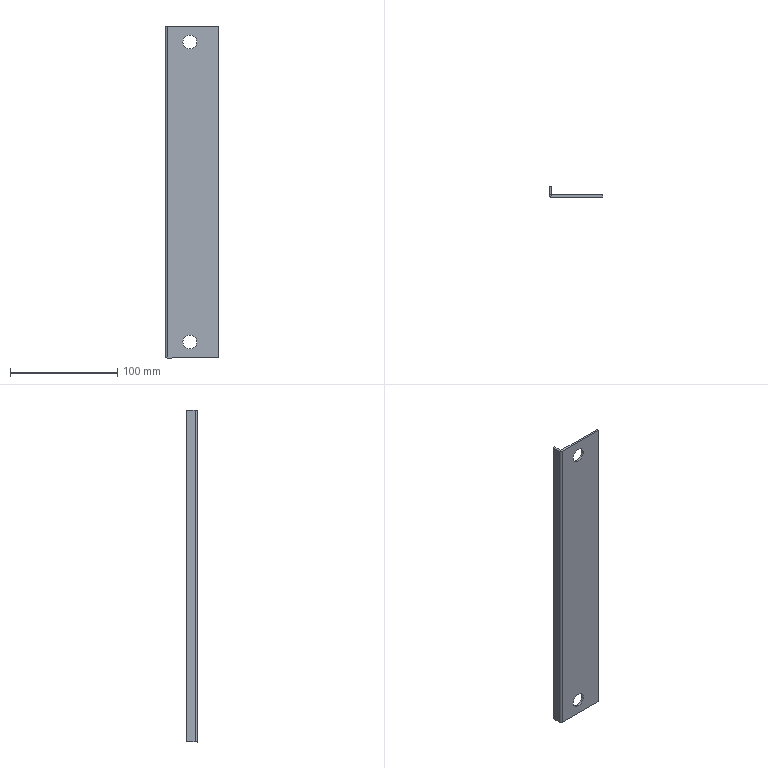Component | SolidWorks | BottomPlateReinforcementBeam-1 | 1 solid | 18 faces | box 50 x 10 x 310 mm | volume 35136 mm3 | plane 12 | cylinder 6 | commonest cylinder face diameters 13 x4 4.2 x1 0.2 x1
STEP:
#1=COLOUR_RGB('',0.7922,0.8196,0.9333);
#2=FILL_AREA_STYLE_COLOUR('',#1);
#3=FILL_AREA_STYLE('',(#2));
#4=SURFACE_STYLE_FILL_AREA(#3);
#5=SURFACE_SIDE_STYLE('',(#4));
#6=SURFACE_STYLE_USAGE(.BOTH.,#5);
#7=PRESENTATION_STYLE_ASSIGNMENT((#6));
#8=CARTESIAN_POINT('',(-12.829,-17.663,36.708));
#9=VERTEX_POINT('',#8);
#10=CARTESIAN_POINT('',(-12.317,-17.663,36.708));
#11=VERTEX_POINT('',#10);
#12=CARTESIAN_POINT('',(-12.573,-17.663,36.708));
#13=DIRECTION('',(0.,1.,-0.));
#14=DIRECTION('',(1.,-0.,0.));
#15=AXIS2_PLACEMENT_3D('',#12,#13,#14);
#16=CIRCLE('',#15,0.2559);
#17=EDGE_CURVE('',#9,#11,#16,.T.);
#18=ORIENTED_EDGE('',*,*,#17,.F.);
#19=CARTESIAN_POINT('',(-12.829,-17.584,36.708));
#20=VERTEX_POINT('',#19);
#21=CARTESIAN_POINT('',(-12.829,-17.978,36.708));
#22=DIRECTION('',(0.,1.,-0.));
#23=VECTOR('',#22,39.37);
#24=LINE('',#21,#23);
#25=EDGE_CURVE('',#9,#20,#24,.T.);
#26=ORIENTED_EDGE('',*,*,#25,.T.);
#27=CARTESIAN_POINT('',(-12.317,-17.584,36.708));
#28=VERTEX_POINT('',#27);
#29=CARTESIAN_POINT('',(-12.573,-17.584,36.708));
#30=DIRECTION('',(0.,1.,-0.));
#31=DIRECTION('',(1.,-0.,0.));
#32=AXIS2_PLACEMENT_3D('',#29,#30,#31);
#33=CIRCLE('',#32,0.2559);
#34=EDGE_CURVE('',#20,#28,#33,.T.);
#35=ORIENTED_EDGE('',*,*,#34,.T.);
#36=CARTESIAN_POINT('',(-12.317,-17.978,36.708));
#37=DIRECTION('',(0.,1.,-0.));
#38=VECTOR('',#37,39.37);
#39=LINE('',#36,#38);
#40=EDGE_CURVE('',#11,#28,#39,.T.);
#41=ORIENTED_EDGE('',*,*,#40,.F.);
#42=EDGE_LOOP('',(#18,#26,#35,#41));
#43=FACE_OUTER_BOUND('',#42,.T.);
#44=CARTESIAN_POINT('',(-12.573,-17.978,36.708));
#45=DIRECTION('',(0.,1.,-0.));
#46=DIRECTION('',(1.,-0.,0.));
#47=AXIS2_PLACEMENT_3D('',#44,#45,#46);
#48=CYLINDRICAL_SURFACE('',#47,0.2559);
#49=ADVANCED_FACE('',(#43),#48,.F.);
#50=CARTESIAN_POINT('',(-12.829,-17.663,25.685));
#51=VERTEX_POINT('',#50);
#52=CARTESIAN_POINT('',(-12.317,-17.663,25.685));
#53=VERTEX_POINT('',#52);
#54=CARTESIAN_POINT('',(-12.573,-17.663,25.685));
#55=DIRECTION('',(0.,1.,-0.));
#56=DIRECTION('',(1.,-0.,0.));
#57=AXIS2_PLACEMENT_3D('',#54,#55,#56);
#58=CIRCLE('',#57,0.2559);
#59=EDGE_CURVE('',#51,#53,#58,.T.);
#60=ORIENTED_EDGE('',*,*,#59,.F.);
#61=CARTESIAN_POINT('',(-12.829,-17.584,25.685));
#62=VERTEX_POINT('',#61);
#63=CARTESIAN_POINT('',(-12.829,-17.978,25.685));
#64=DIRECTION('',(0.,1.,-0.));
#65=VECTOR('',#64,39.37);
#66=LINE('',#63,#65);
#67=EDGE_CURVE('',#51,#62,#66,.T.);
#68=ORIENTED_EDGE('',*,*,#67,.T.);
#69=CARTESIAN_POINT('',(-12.317,-17.584,25.685));
#70=VERTEX_POINT('',#69);
#71=CARTESIAN_POINT('',(-12.573,-17.584,25.685));
#72=DIRECTION('',(0.,1.,-0.));
#73=DIRECTION('',(1.,-0.,0.));
#74=AXIS2_PLACEMENT_3D('',#71,#72,#73);
#75=CIRCLE('',#74,0.2559);
#76=EDGE_CURVE('',#62,#70,#75,.T.);
#77=ORIENTED_EDGE('',*,*,#76,.T.);
#78=CARTESIAN_POINT('',(-12.317,-17.978,25.685));
#79=DIRECTION('',(0.,1.,-0.));
#80=VECTOR('',#79,39.37);
#81=LINE('',#78,#80);
#82=EDGE_CURVE('',#53,#70,#81,.T.);
#83=ORIENTED_EDGE('',*,*,#82,.F.);
#84=EDGE_LOOP('',(#60,#68,#77,#83));
#85=FACE_OUTER_BOUND('',#84,.T.);
#86=CARTESIAN_POINT('',(-12.573,-17.978,25.685));
#87=DIRECTION('',(0.,1.,-0.));
#88=DIRECTION('',(1.,-0.,0.));
#89=AXIS2_PLACEMENT_3D('',#86,#87,#88);
#90=CYLINDRICAL_SURFACE('',#89,0.2559);
#91=ADVANCED_FACE('',(#85),#90,.F.);
#92=CARTESIAN_POINT('',(-13.396,-17.584,37.299));
#93=VERTEX_POINT('',#92);
#94=CARTESIAN_POINT('',(-11.51,-17.584,37.299));
#95=VERTEX_POINT('',#94);
#96=CARTESIAN_POINT('',(-13.479,-17.584,37.299));
#97=DIRECTION('',(1.,-0.,0.));
#98=VECTOR('',#97,39.37);
#99=LINE('',#96,#98);
#100=EDGE_CURVE('',#93,#95,#99,.T.);
#101=ORIENTED_EDGE('',*,*,#100,.F.);
#102=CARTESIAN_POINT('',(-13.396,-17.663,37.299));
#103=VERTEX_POINT('',#102);
#104=CARTESIAN_POINT('',(-13.396,-17.584,37.299));
#105=DIRECTION('',(0.,-1.,0.));
#106=VECTOR('',#105,39.37);
#107=LINE('',#104,#106);
#108=EDGE_CURVE('',#93,#103,#107,.T.);
#109=ORIENTED_EDGE('',*,*,#108,.T.);
#110=CARTESIAN_POINT('',(-11.51,-17.663,37.299));
#111=VERTEX_POINT('',#110);
#112=CARTESIAN_POINT('',(-13.479,-17.663,37.299));
#113=DIRECTION('',(1.,-0.,0.));
#114=VECTOR('',#113,39.37);
#115=LINE('',#112,#114);
#116=EDGE_CURVE('',#103,#111,#115,.T.);
#117=ORIENTED_EDGE('',*,*,#116,.T.);
#118=CARTESIAN_POINT('',(-11.51,-17.663,37.299));
#119=DIRECTION('',(0.,1.,-0.));
#120=VECTOR('',#119,39.37);
#121=LINE('',#118,#120);
#122=EDGE_CURVE('',#111,#95,#121,.T.);
#123=ORIENTED_EDGE('',*,*,#122,.T.);
#124=EDGE_LOOP('',(#101,#109,#117,#123));
#125=FACE_OUTER_BOUND('',#124,.T.);
#126=CARTESIAN_POINT('',(-13.479,-17.663,37.299));
#127=DIRECTION('',(-0.,0.,1.));
#128=DIRECTION('',(-0.,-1.,0.));
#129=AXIS2_PLACEMENT_3D('',#126,#127,#128);
#130=PLANE('',#129);
#131=ADVANCED_FACE('',(#125),#130,.T.);
#132=CARTESIAN_POINT('',(-12.573,-17.663,25.685));
#133=DIRECTION('',(0.,1.,-0.));
#134=DIRECTION('',(1.,-0.,0.));
#135=AXIS2_PLACEMENT_3D('',#132,#133,#134);
#136=CIRCLE('',#135,0.2559);
#137=EDGE_CURVE('',#53,#51,#136,.T.);
#138=ORIENTED_EDGE('',*,*,#137,.T.);
#139=ORIENTED_EDGE('',*,*,#59,.T.);
#140=EDGE_LOOP('',(#138,#139));
#141=FACE_BOUND('',#140,.T.);
#142=CARTESIAN_POINT('',(-12.573,-17.663,36.708));
#143=DIRECTION('',(0.,1.,-0.));
#144=DIRECTION('',(1.,-0.,0.));
#145=AXIS2_PLACEMENT_3D('',#142,#143,#144);
#146=CIRCLE('',#145,0.2559);
#147=EDGE_CURVE('',#11,#9,#146,.T.);
#148=ORIENTED_EDGE('',*,*,#147,.T.);
#149=ORIENTED_EDGE('',*,*,#17,.T.);
#150=EDGE_LOOP('',(#148,#149));
#151=FACE_BOUND('',#150,.T.);
#152=CARTESIAN_POINT('',(-13.396,-17.663,25.094));
#153=VERTEX_POINT('',#152);
#154=CARTESIAN_POINT('',(-13.396,-17.663,37.299));
#155=DIRECTION('',(0.,-0.,-1.));
#156=VECTOR('',#155,39.37);
#157=LINE('',#154,#156);
#158=EDGE_CURVE('',#103,#153,#157,.T.);
#159=ORIENTED_EDGE('',*,*,#158,.T.);
#160=CARTESIAN_POINT('',(-11.51,-17.663,25.094));
#161=VERTEX_POINT('',#160);
#162=CARTESIAN_POINT('',(-13.479,-17.663,25.094));
#163=DIRECTION('',(-1.,0.,-0.));
#164=VECTOR('',#163,39.37);
#165=LINE('',#162,#164);
#166=EDGE_CURVE('',#161,#153,#165,.T.);
#167=ORIENTED_EDGE('',*,*,#166,.F.);
#168=CARTESIAN_POINT('',(-11.51,-17.663,25.094));
#169=DIRECTION('',(0.,-0.,-1.));
#170=VECTOR('',#169,39.37);
#171=LINE('',#168,#170);
#172=EDGE_CURVE('',#111,#161,#171,.T.);
#173=ORIENTED_EDGE('',*,*,#172,.F.);
#174=ORIENTED_EDGE('',*,*,#116,.F.);
#175=EDGE_LOOP('',(#159,#167,#173,#174));
#176=FACE_OUTER_BOUND('',#175,.T.);
#177=CARTESIAN_POINT('',(-12.494,-17.663,31.196));
#178=DIRECTION('',(0.,1.,-0.));
#179=DIRECTION('',(1.,-0.,0.));
#180=AXIS2_PLACEMENT_3D('',#177,#178,#179);
#181=PLANE('',#180);
#182=ADVANCED_FACE('',(#141,#151,#176),#181,.F.);
#183=CARTESIAN_POINT('',(-12.573,-17.584,36.708));
#184=DIRECTION('',(0.,1.,-0.));
#185=DIRECTION('',(1.,-0.,0.));
#186=AXIS2_PLACEMENT_3D('',#183,#184,#185);
#187=CIRCLE('',#186,0.2559);
#188=EDGE_CURVE('',#28,#20,#187,.T.);
#189=ORIENTED_EDGE('',*,*,#188,.F.);
#190=ORIENTED_EDGE('',*,*,#34,.F.);
#191=EDGE_LOOP('',(#189,#190));
#192=FACE_BOUND('',#191,.T.);
#193=CARTESIAN_POINT('',(-12.573,-17.584,25.685));
#194=DIRECTION('',(0.,1.,-0.));
#195=DIRECTION('',(1.,-0.,0.));
#196=AXIS2_PLACEMENT_3D('',#193,#194,#195);
#197=CIRCLE('',#196,0.2559);
#198=EDGE_CURVE('',#70,#62,#197,.T.);
#199=ORIENTED_EDGE('',*,*,#198,.F.);
#200=ORIENTED_EDGE('',*,*,#76,.F.);
#201=EDGE_LOOP('',(#199,#200));
#202=FACE_BOUND('',#201,.T.);
#203=CARTESIAN_POINT('',(-11.51,-17.584,25.094));
#204=VERTEX_POINT('',#203);
#205=CARTESIAN_POINT('',(-13.396,-17.584,25.094));
#206=VERTEX_POINT('',#205);
#207=CARTESIAN_POINT('',(-13.479,-17.584,25.094));
#208=DIRECTION('',(-1.,0.,-0.));
#209=VECTOR('',#208,39.37);
#210=LINE('',#207,#209);
#211=EDGE_CURVE('',#204,#206,#210,.T.);
#212=ORIENTED_EDGE('',*,*,#211,.T.);
#213=CARTESIAN_POINT('',(-13.396,-17.584,37.299));
#214=DIRECTION('',(0.,-0.,-1.));
#215=VECTOR('',#214,39.37);
#216=LINE('',#213,#215);
#217=EDGE_CURVE('',#93,#206,#216,.T.);
#218=ORIENTED_EDGE('',*,*,#217,.F.);
#219=ORIENTED_EDGE('',*,*,#100,.T.);
#220=CARTESIAN_POINT('',(-11.51,-17.584,25.094));
#221=DIRECTION('',(0.,-0.,-1.));
#222=VECTOR('',#221,39.37);
#223=LINE('',#220,#222);
#224=EDGE_CURVE('',#95,#204,#223,.T.);
#225=ORIENTED_EDGE('',*,*,#224,.T.);
#226=EDGE_LOOP('',(#212,#218,#219,#225));
#227=FACE_OUTER_BOUND('',#226,.T.);
#228=CARTESIAN_POINT('',(-12.494,-17.584,31.196));
#229=DIRECTION('',(0.,1.,-0.));
#230=DIRECTION('',(1.,-0.,0.));
#231=AXIS2_PLACEMENT_3D('',#228,#229,#230);
#232=PLANE('',#231);
#233=ADVANCED_FACE('',(#192,#202,#227),#232,.T.);
#234=ORIENTED_EDGE('',*,*,#224,.F.);
#235=ORIENTED_EDGE('',*,*,#122,.F.);
#236=ORIENTED_EDGE('',*,*,#172,.T.);
#237=CARTESIAN_POINT('',(-11.51,-17.663,25.094));
#238=DIRECTION('',(0.,1.,-0.));
#239=VECTOR('',#238,39.37);
#240=LINE('',#237,#239);
#241=EDGE_CURVE('',#161,#204,#240,.T.);
#242=ORIENTED_EDGE('',*,*,#241,.T.);
#243=EDGE_LOOP('',(#234,#235,#236,#242));
#244=FACE_OUTER_BOUND('',#243,.T.);
#245=CARTESIAN_POINT('',(-11.51,-17.663,25.094));
#246=DIRECTION('',(1.,-0.,0.));
#247=DIRECTION('',(0.,-0.,-1.));
#248=AXIS2_PLACEMENT_3D('',#245,#246,#247);
#249=PLANE('',#248);
#250=ADVANCED_FACE('',(#244),#249,.T.);
#251=CARTESIAN_POINT('',(-13.396,-17.584,25.094));
#252=DIRECTION('',(0.,-1.,0.));
#253=VECTOR('',#252,39.37);
#254=LINE('',#251,#253);
#255=EDGE_CURVE('',#206,#153,#254,.T.);
#256=ORIENTED_EDGE('',*,*,#255,.F.);
#257=ORIENTED_EDGE('',*,*,#211,.F.);
#258=ORIENTED_EDGE('',*,*,#241,.F.);
#259=ORIENTED_EDGE('',*,*,#166,.T.);
#260=EDGE_LOOP('',(#256,#257,#258,#259));
#261=FACE_OUTER_BOUND('',#260,.T.);
#262=CARTESIAN_POINT('',(-13.479,-17.663,25.094));
#263=DIRECTION('',(0.,-0.,-1.));
#264=DIRECTION('',(0.,1.,-0.));
#265=AXIS2_PLACEMENT_3D('',#262,#263,#264);
#266=PLANE('',#265);
#267=ADVANCED_FACE('',(#261),#266,.T.);
#268=ORIENTED_EDGE('',*,*,#67,.F.);
#269=ORIENTED_EDGE('',*,*,#137,.F.);
#270=ORIENTED_EDGE('',*,*,#82,.T.);
#271=ORIENTED_EDGE('',*,*,#198,.T.);
#272=EDGE_LOOP('',(#268,#269,#270,#271));
#273=FACE_OUTER_BOUND('',#272,.T.);
#274=CARTESIAN_POINT('',(-12.573,-17.978,25.685));
#275=DIRECTION('',(0.,1.,-0.));
#276=DIRECTION('',(1.,-0.,0.));
#277=AXIS2_PLACEMENT_3D('',#274,#275,#276);
#278=CYLINDRICAL_SURFACE('',#277,0.2559);
#279=ADVANCED_FACE('',(#273),#278,.F.);
#280=ORIENTED_EDGE('',*,*,#25,.F.);
#281=ORIENTED_EDGE('',*,*,#147,.F.);
#282=ORIENTED_EDGE('',*,*,#40,.T.);
#283=ORIENTED_EDGE('',*,*,#188,.T.);
#284=EDGE_LOOP('',(#280,#281,#282,#283));
#285=FACE_OUTER_BOUND('',#284,.T.);
#286=CARTESIAN_POINT('',(-12.573,-17.978,36.708));
#287=DIRECTION('',(0.,1.,-0.));
#288=DIRECTION('',(1.,-0.,0.));
#289=AXIS2_PLACEMENT_3D('',#286,#287,#288);
#290=CYLINDRICAL_SURFACE('',#289,0.2559);
#291=ADVANCED_FACE('',(#285),#290,.F.);
#292=CARTESIAN_POINT('',(-13.4,-17.58,25.094));
#293=VERTEX_POINT('',#292);
#294=CARTESIAN_POINT('',(-13.479,-17.58,25.094));
#295=VERTEX_POINT('',#294);
#296=CARTESIAN_POINT('',(-13.479,-17.58,25.094));
#297=DIRECTION('',(-1.,0.,-0.));
#298=VECTOR('',#297,39.37);
#299=LINE('',#296,#298);
#300=EDGE_CURVE('',#293,#295,#299,.T.);
#301=ORIENTED_EDGE('',*,*,#300,.F.);
#302=CARTESIAN_POINT('',(-13.396,-17.58,25.094));
#303=DIRECTION('',(0.,-0.,-1.));
#304=DIRECTION('',(0.,-1.,0.));
#305=AXIS2_PLACEMENT_3D('',#302,#303,#304);
#306=CIRCLE('',#305,0.003937);
#307=EDGE_CURVE('',#206,#293,#306,.T.);
#308=ORIENTED_EDGE('',*,*,#307,.F.);
#309=ORIENTED_EDGE('',*,*,#255,.T.);
#310=CARTESIAN_POINT('',(-13.396,-17.58,25.094));
#311=DIRECTION('',(0.,-0.,-1.));
#312=DIRECTION('',(0.,-1.,0.));
#313=AXIS2_PLACEMENT_3D('',#310,#311,#312);
#314=CIRCLE('',#313,0.08268);
#315=EDGE_CURVE('',#153,#295,#314,.T.);
#316=ORIENTED_EDGE('',*,*,#315,.T.);
#317=EDGE_LOOP('',(#301,#308,#309,#316));
#318=FACE_OUTER_BOUND('',#317,.T.);
#319=CARTESIAN_POINT('',(-13.396,-17.58,25.094));
#320=DIRECTION('',(0.,-0.,-1.));
#321=DIRECTION('',(0.,1.,-0.));
#322=AXIS2_PLACEMENT_3D('',#319,#320,#321);
#323=PLANE('',#322);
#324=ADVANCED_FACE('',(#318),#323,.T.);
#325=CARTESIAN_POINT('',(-13.4,-17.58,37.299));
#326=VERTEX_POINT('',#325);
#327=CARTESIAN_POINT('',(-13.396,-17.58,37.299));
#328=DIRECTION('',(-0.,0.,1.));
#329=DIRECTION('',(0.,-1.,0.));
#330=AXIS2_PLACEMENT_3D('',#327,#328,#329);
#331=CIRCLE('',#330,0.003937);
#332=EDGE_CURVE('',#326,#93,#331,.T.);
#333=ORIENTED_EDGE('',*,*,#332,.F.);
#334=CARTESIAN_POINT('',(-13.479,-17.58,37.299));
#335=VERTEX_POINT('',#334);
#336=CARTESIAN_POINT('',(-13.4,-17.58,37.299));
#337=DIRECTION('',(-1.,0.,-0.));
#338=VECTOR('',#337,39.37);
#339=LINE('',#336,#338);
#340=EDGE_CURVE('',#326,#335,#339,.T.);
#341=ORIENTED_EDGE('',*,*,#340,.T.);
#342=CARTESIAN_POINT('',(-13.396,-17.58,37.299));
#343=DIRECTION('',(-0.,0.,1.));
#344=DIRECTION('',(0.,-1.,0.));
#345=AXIS2_PLACEMENT_3D('',#342,#343,#344);
#346=CIRCLE('',#345,0.08268);
#347=EDGE_CURVE('',#335,#103,#346,.T.);
#348=ORIENTED_EDGE('',*,*,#347,.T.);
#349=ORIENTED_EDGE('',*,*,#108,.F.);
#350=EDGE_LOOP('',(#333,#341,#348,#349));
#351=FACE_OUTER_BOUND('',#350,.T.);
#352=CARTESIAN_POINT('',(-13.396,-17.58,37.299));
#353=DIRECTION('',(0.,-0.,-1.));
#354=DIRECTION('',(0.,1.,-0.));
#355=AXIS2_PLACEMENT_3D('',#352,#353,#354);
#356=PLANE('',#355);
#357=ADVANCED_FACE('',(#351),#356,.F.);
#358=ORIENTED_EDGE('',*,*,#158,.F.);
#359=ORIENTED_EDGE('',*,*,#347,.F.);
#360=CARTESIAN_POINT('',(-13.479,-17.58,25.094));
#361=DIRECTION('',(0.,-0.,-1.));
#362=VECTOR('',#361,39.37);
#363=LINE('',#360,#362);
#364=EDGE_CURVE('',#335,#295,#363,.T.);
#365=ORIENTED_EDGE('',*,*,#364,.T.);
#366=ORIENTED_EDGE('',*,*,#315,.F.);
#367=EDGE_LOOP('',(#358,#359,#365,#366));
#368=FACE_OUTER_BOUND('',#367,.T.);
#369=CARTESIAN_POINT('',(-13.396,-17.58,37.299));
#370=DIRECTION('',(-0.,0.,1.));
#371=DIRECTION('',(-1.,0.,0.));
#372=AXIS2_PLACEMENT_3D('',#369,#370,#371);
#373=CYLINDRICAL_SURFACE('',#372,0.08268);
#374=ADVANCED_FACE('',(#368),#373,.T.);
#375=ORIENTED_EDGE('',*,*,#217,.T.);
#376=ORIENTED_EDGE('',*,*,#307,.T.);
#377=CARTESIAN_POINT('',(-13.4,-17.58,25.094));
#378=DIRECTION('',(-0.,0.,1.));
#379=VECTOR('',#378,39.37);
#380=LINE('',#377,#379);
#381=EDGE_CURVE('',#293,#326,#380,.T.);
#382=ORIENTED_EDGE('',*,*,#381,.T.);
#383=ORIENTED_EDGE('',*,*,#332,.T.);
#384=EDGE_LOOP('',(#375,#376,#382,#383));
#385=FACE_OUTER_BOUND('',#384,.T.);
#386=CARTESIAN_POINT('',(-13.396,-17.58,37.299));
#387=DIRECTION('',(-0.,0.,1.));
#388=DIRECTION('',(-1.,0.,0.));
#389=AXIS2_PLACEMENT_3D('',#386,#387,#388);
#390=CYLINDRICAL_SURFACE('',#389,0.003937);
#391=ADVANCED_FACE('',(#385),#390,.F.);
#392=ORIENTED_EDGE('',*,*,#340,.F.);
#393=CARTESIAN_POINT('',(-13.4,-17.269,37.299));
#394=VERTEX_POINT('',#393);
#395=CARTESIAN_POINT('',(-13.4,-17.269,37.299));
#396=DIRECTION('',(0.,1.,-0.));
#397=VECTOR('',#396,39.37);
#398=LINE('',#395,#397);
#399=EDGE_CURVE('',#326,#394,#398,.T.);
#400=ORIENTED_EDGE('',*,*,#399,.T.);
#401=CARTESIAN_POINT('',(-13.479,-17.269,37.299));
#402=VERTEX_POINT('',#401);
#403=CARTESIAN_POINT('',(-13.479,-17.269,37.299));
#404=DIRECTION('',(1.,-0.,0.));
#405=VECTOR('',#404,39.37);
#406=LINE('',#403,#405);
#407=EDGE_CURVE('',#402,#394,#406,.T.);
#408=ORIENTED_EDGE('',*,*,#407,.F.);
#409=CARTESIAN_POINT('',(-13.479,-17.584,37.299));
#410=DIRECTION('',(0.,1.,-0.));
#411=VECTOR('',#410,39.37);
#412=LINE('',#409,#411);
#413=EDGE_CURVE('',#335,#402,#412,.T.);
#414=ORIENTED_EDGE('',*,*,#413,.F.);
#415=EDGE_LOOP('',(#392,#400,#408,#414));
#416=FACE_OUTER_BOUND('',#415,.T.);
#417=CARTESIAN_POINT('',(-13.479,-17.269,37.299));
#418=DIRECTION('',(0.,-0.,-1.));
#419=DIRECTION('',(-1.,0.,-0.));
#420=AXIS2_PLACEMENT_3D('',#417,#418,#419);
#421=PLANE('',#420);
#422=ADVANCED_FACE('',(#416),#421,.F.);
#423=ORIENTED_EDGE('',*,*,#300,.T.);
#424=CARTESIAN_POINT('',(-13.479,-17.269,25.094));
#425=VERTEX_POINT('',#424);
#426=CARTESIAN_POINT('',(-13.479,-17.584,25.094));
#427=DIRECTION('',(-0.,-1.,0.));
#428=VECTOR('',#427,39.37);
#429=LINE('',#426,#428);
#430=EDGE_CURVE('',#425,#295,#429,.T.);
#431=ORIENTED_EDGE('',*,*,#430,.F.);
#432=CARTESIAN_POINT('',(-13.4,-17.269,25.094));
#433=VERTEX_POINT('',#432);
#434=CARTESIAN_POINT('',(-13.479,-17.269,25.094));
#435=DIRECTION('',(1.,-0.,0.));
#436=VECTOR('',#435,39.37);
#437=LINE('',#434,#436);
#438=EDGE_CURVE('',#425,#433,#437,.T.);
#439=ORIENTED_EDGE('',*,*,#438,.T.);
#440=CARTESIAN_POINT('',(-13.4,-17.584,25.094));
#441=DIRECTION('',(-0.,-1.,0.));
#442=VECTOR('',#441,39.37);
#443=LINE('',#440,#442);
#444=EDGE_CURVE('',#433,#293,#443,.T.);
#445=ORIENTED_EDGE('',*,*,#444,.T.);
#446=EDGE_LOOP('',(#423,#431,#439,#445));
#447=FACE_OUTER_BOUND('',#446,.T.);
#448=CARTESIAN_POINT('',(-13.479,-17.584,25.094));
#449=DIRECTION('',(-0.,0.,1.));
#450=DIRECTION('',(1.,-0.,0.));
#451=AXIS2_PLACEMENT_3D('',#448,#449,#450);
#452=PLANE('',#451);
#453=ADVANCED_FACE('',(#447),#452,.F.);
#454=ORIENTED_EDGE('',*,*,#364,.F.);
#455=ORIENTED_EDGE('',*,*,#413,.T.);
#456=CARTESIAN_POINT('',(-13.479,-17.269,31.196));
#457=DIRECTION('',(0.,-0.,-1.));
#458=VECTOR('',#457,39.37);
#459=LINE('',#456,#458);
#460=EDGE_CURVE('',#402,#425,#459,.T.);
#461=ORIENTED_EDGE('',*,*,#460,.T.);
#462=ORIENTED_EDGE('',*,*,#430,.T.);
#463=EDGE_LOOP('',(#454,#455,#461,#462));
#464=FACE_OUTER_BOUND('',#463,.T.);
#465=CARTESIAN_POINT('',(-13.479,-17.584,31.196));
#466=DIRECTION('',(1.,-0.,0.));
#467=DIRECTION('',(-0.,-1.,0.));
#468=AXIS2_PLACEMENT_3D('',#465,#466,#467);
#469=PLANE('',#468);
#470=ADVANCED_FACE('',(#464),#469,.F.);
#471=ORIENTED_EDGE('',*,*,#399,.F.);
#472=ORIENTED_EDGE('',*,*,#381,.F.);
#473=ORIENTED_EDGE('',*,*,#444,.F.);
#474=CARTESIAN_POINT('',(-13.4,-17.269,25.094));
#475=DIRECTION('',(0.,-0.,-1.));
#476=VECTOR('',#475,39.37);
#477=LINE('',#474,#476);
#478=EDGE_CURVE('',#394,#433,#477,.T.);
#479=ORIENTED_EDGE('',*,*,#478,.F.);
#480=EDGE_LOOP('',(#471,#472,#473,#479));
#481=FACE_OUTER_BOUND('',#480,.T.);
#482=CARTESIAN_POINT('',(-13.4,-17.584,31.196));
#483=DIRECTION('',(1.,-0.,0.));
#484=DIRECTION('',(-0.,-1.,0.));
#485=AXIS2_PLACEMENT_3D('',#482,#483,#484);
#486=PLANE('',#485);
#487=ADVANCED_FACE('',(#481),#486,.T.);
#488=ORIENTED_EDGE('',*,*,#478,.T.);
#489=ORIENTED_EDGE('',*,*,#438,.F.);
#490=ORIENTED_EDGE('',*,*,#460,.F.);
#491=ORIENTED_EDGE('',*,*,#407,.T.);
#492=EDGE_LOOP('',(#488,#489,#490,#491));
#493=FACE_OUTER_BOUND('',#492,.T.);
#494=CARTESIAN_POINT('',(-13.479,-17.269,25.094));
#495=DIRECTION('',(-0.,-1.,0.));
#496=DIRECTION('',(-1.,0.,-0.));
#497=AXIS2_PLACEMENT_3D('',#494,#495,#496);
#498=PLANE('',#497);
#499=ADVANCED_FACE('',(#493),#498,.F.);
#500=CLOSED_SHELL('',(#49,#91,#131,#182,#233,#250,#267,#279,#291,#324,#357,#374,#391,#422,#453,#470,#487,#499));
#501=MANIFOLD_SOLID_BREP('',#500);
#502=STYLED_ITEM('',(#7),#501);
#503=(LENGTH_UNIT()NAMED_UNIT(*)SI_UNIT($,.METRE.));
#504=LENGTH_MEASURE_WITH_UNIT(LENGTH_MEASURE(0.0254),#503);
#505=DIMENSIONAL_EXPONENTS(1.,0.,0.,0.,0.,0.,0.);
#506=(CONVERSION_BASED_UNIT('',#504)LENGTH_UNIT()NAMED_UNIT(#505));
#507=UNCERTAINTY_MEASURE_WITH_UNIT(LENGTH_MEASURE(0.00001),#506,'','');
#508=(NAMED_UNIT(*)PLANE_ANGLE_UNIT()SI_UNIT($,.RADIAN.));
#509=(NAMED_UNIT(*)SI_UNIT($,.STERADIAN.)SOLID_ANGLE_UNIT());
#510=(GEOMETRIC_REPRESENTATION_CONTEXT(3)GLOBAL_UNCERTAINTY_ASSIGNED_CONTEXT((#507))GLOBAL_UNIT_ASSIGNED_CONTEXT((#506,#508,#509))REPRESENTATION_CONTEXT('',''));
#511=MECHANICAL_DESIGN_GEOMETRIC_PRESENTATION_REPRESENTATION('',(#502),#510);
#512=PRESENTATION_LAYER_ASSIGNMENT('','',(#502));
#513=CARTESIAN_POINT('',(0.,0.,0.));
#514=DIRECTION('',(0.,0.,1.));
#515=DIRECTION('',(1.,0.,0.));
#516=AXIS2_PLACEMENT_3D('',#513,#514,#515);
#517=(LENGTH_UNIT()NAMED_UNIT(*)SI_UNIT($,.METRE.));
#518=LENGTH_MEASURE_WITH_UNIT(LENGTH_MEASURE(0.0254),#517);
#519=DIMENSIONAL_EXPONENTS(1.,0.,0.,0.,0.,0.,0.);
#520=(CONVERSION_BASED_UNIT('',#518)LENGTH_UNIT()NAMED_UNIT(#519));
#521=UNCERTAINTY_MEASURE_WITH_UNIT(LENGTH_MEASURE(0.00001),#520,'','');
#522=(NAMED_UNIT(*)PLANE_ANGLE_UNIT()SI_UNIT($,.RADIAN.));
#523=(NAMED_UNIT(*)SI_UNIT($,.STERADIAN.)SOLID_ANGLE_UNIT());
#524=(GEOMETRIC_REPRESENTATION_CONTEXT(3)GLOBAL_UNCERTAINTY_ASSIGNED_CONTEXT((#521))GLOBAL_UNIT_ASSIGNED_CONTEXT((#520,#522,#523))REPRESENTATION_CONTEXT('',''));
#525=ADVANCED_BREP_SHAPE_REPRESENTATION('',(#501,#516),#524);